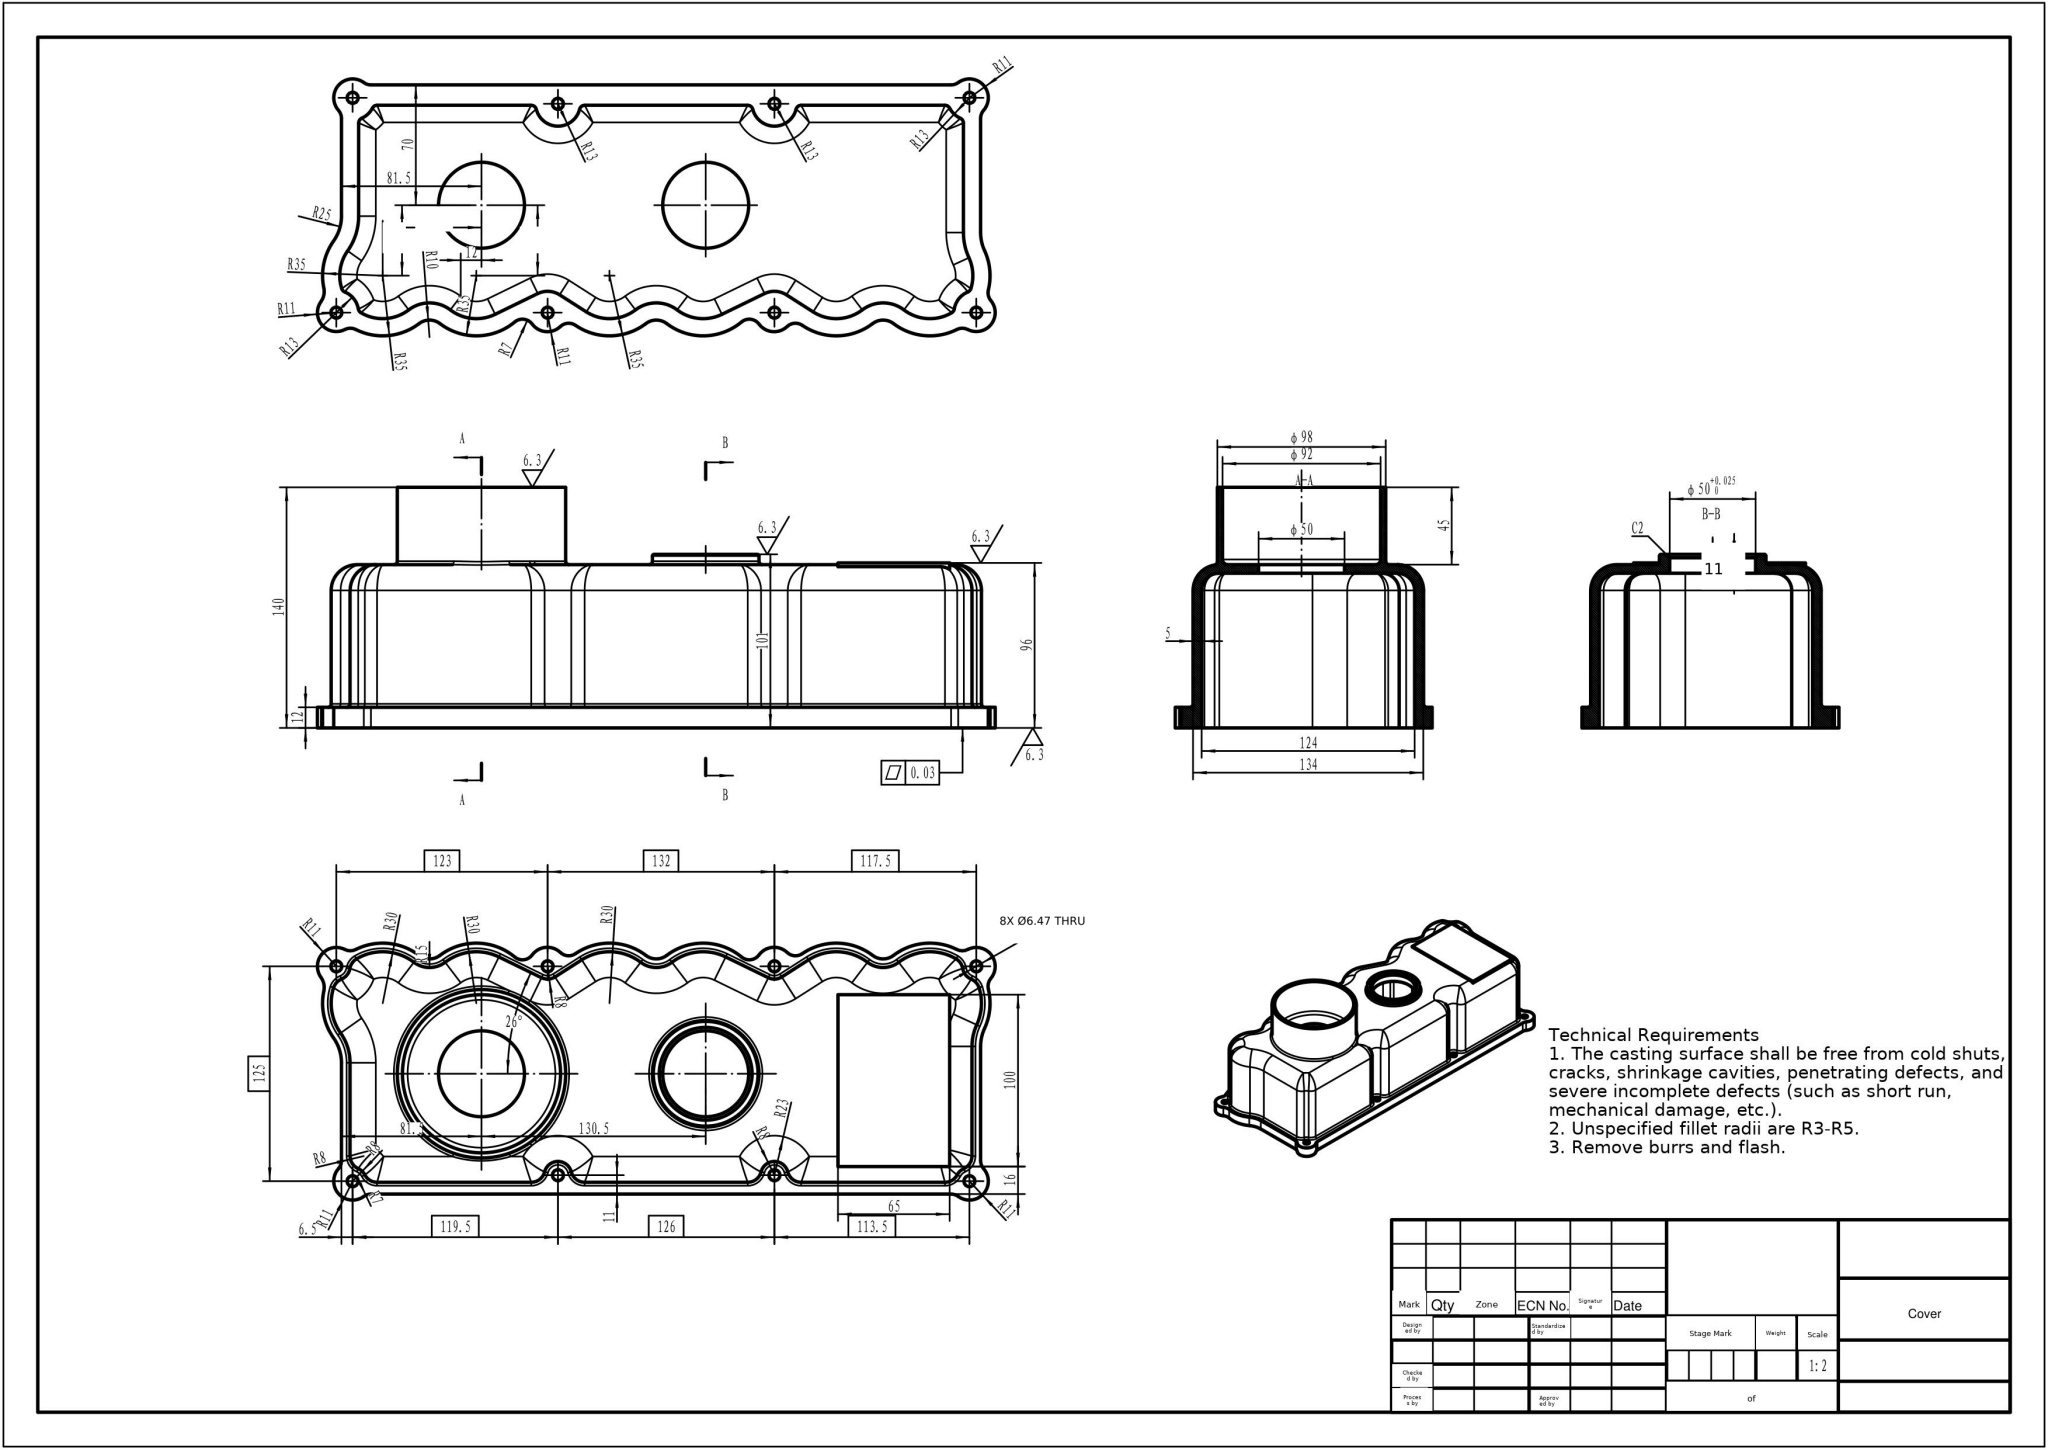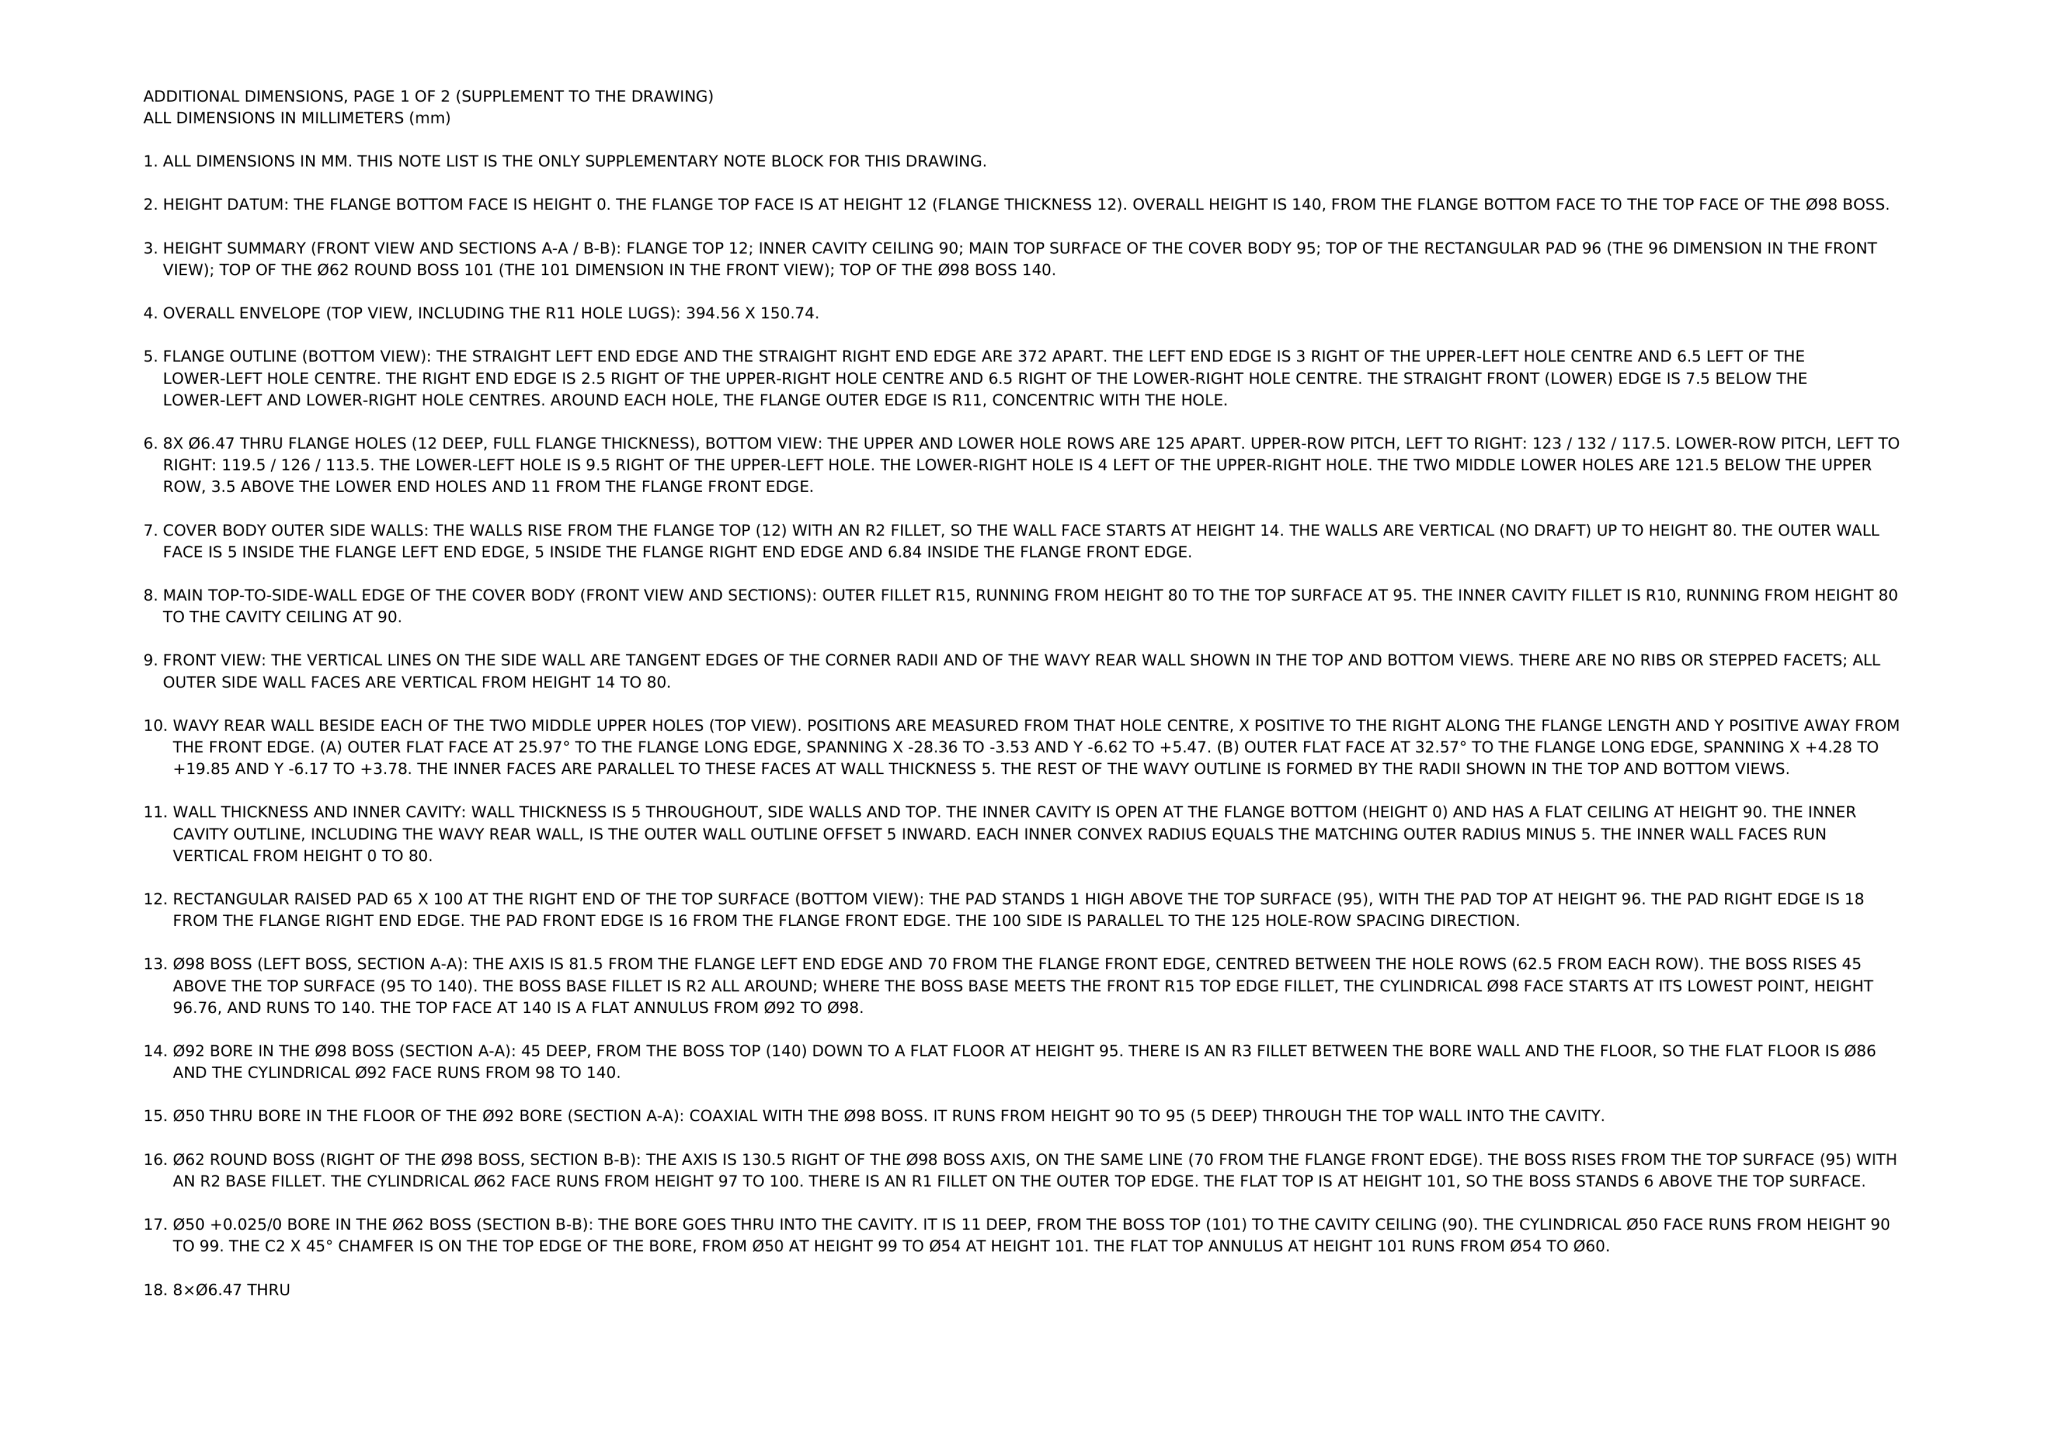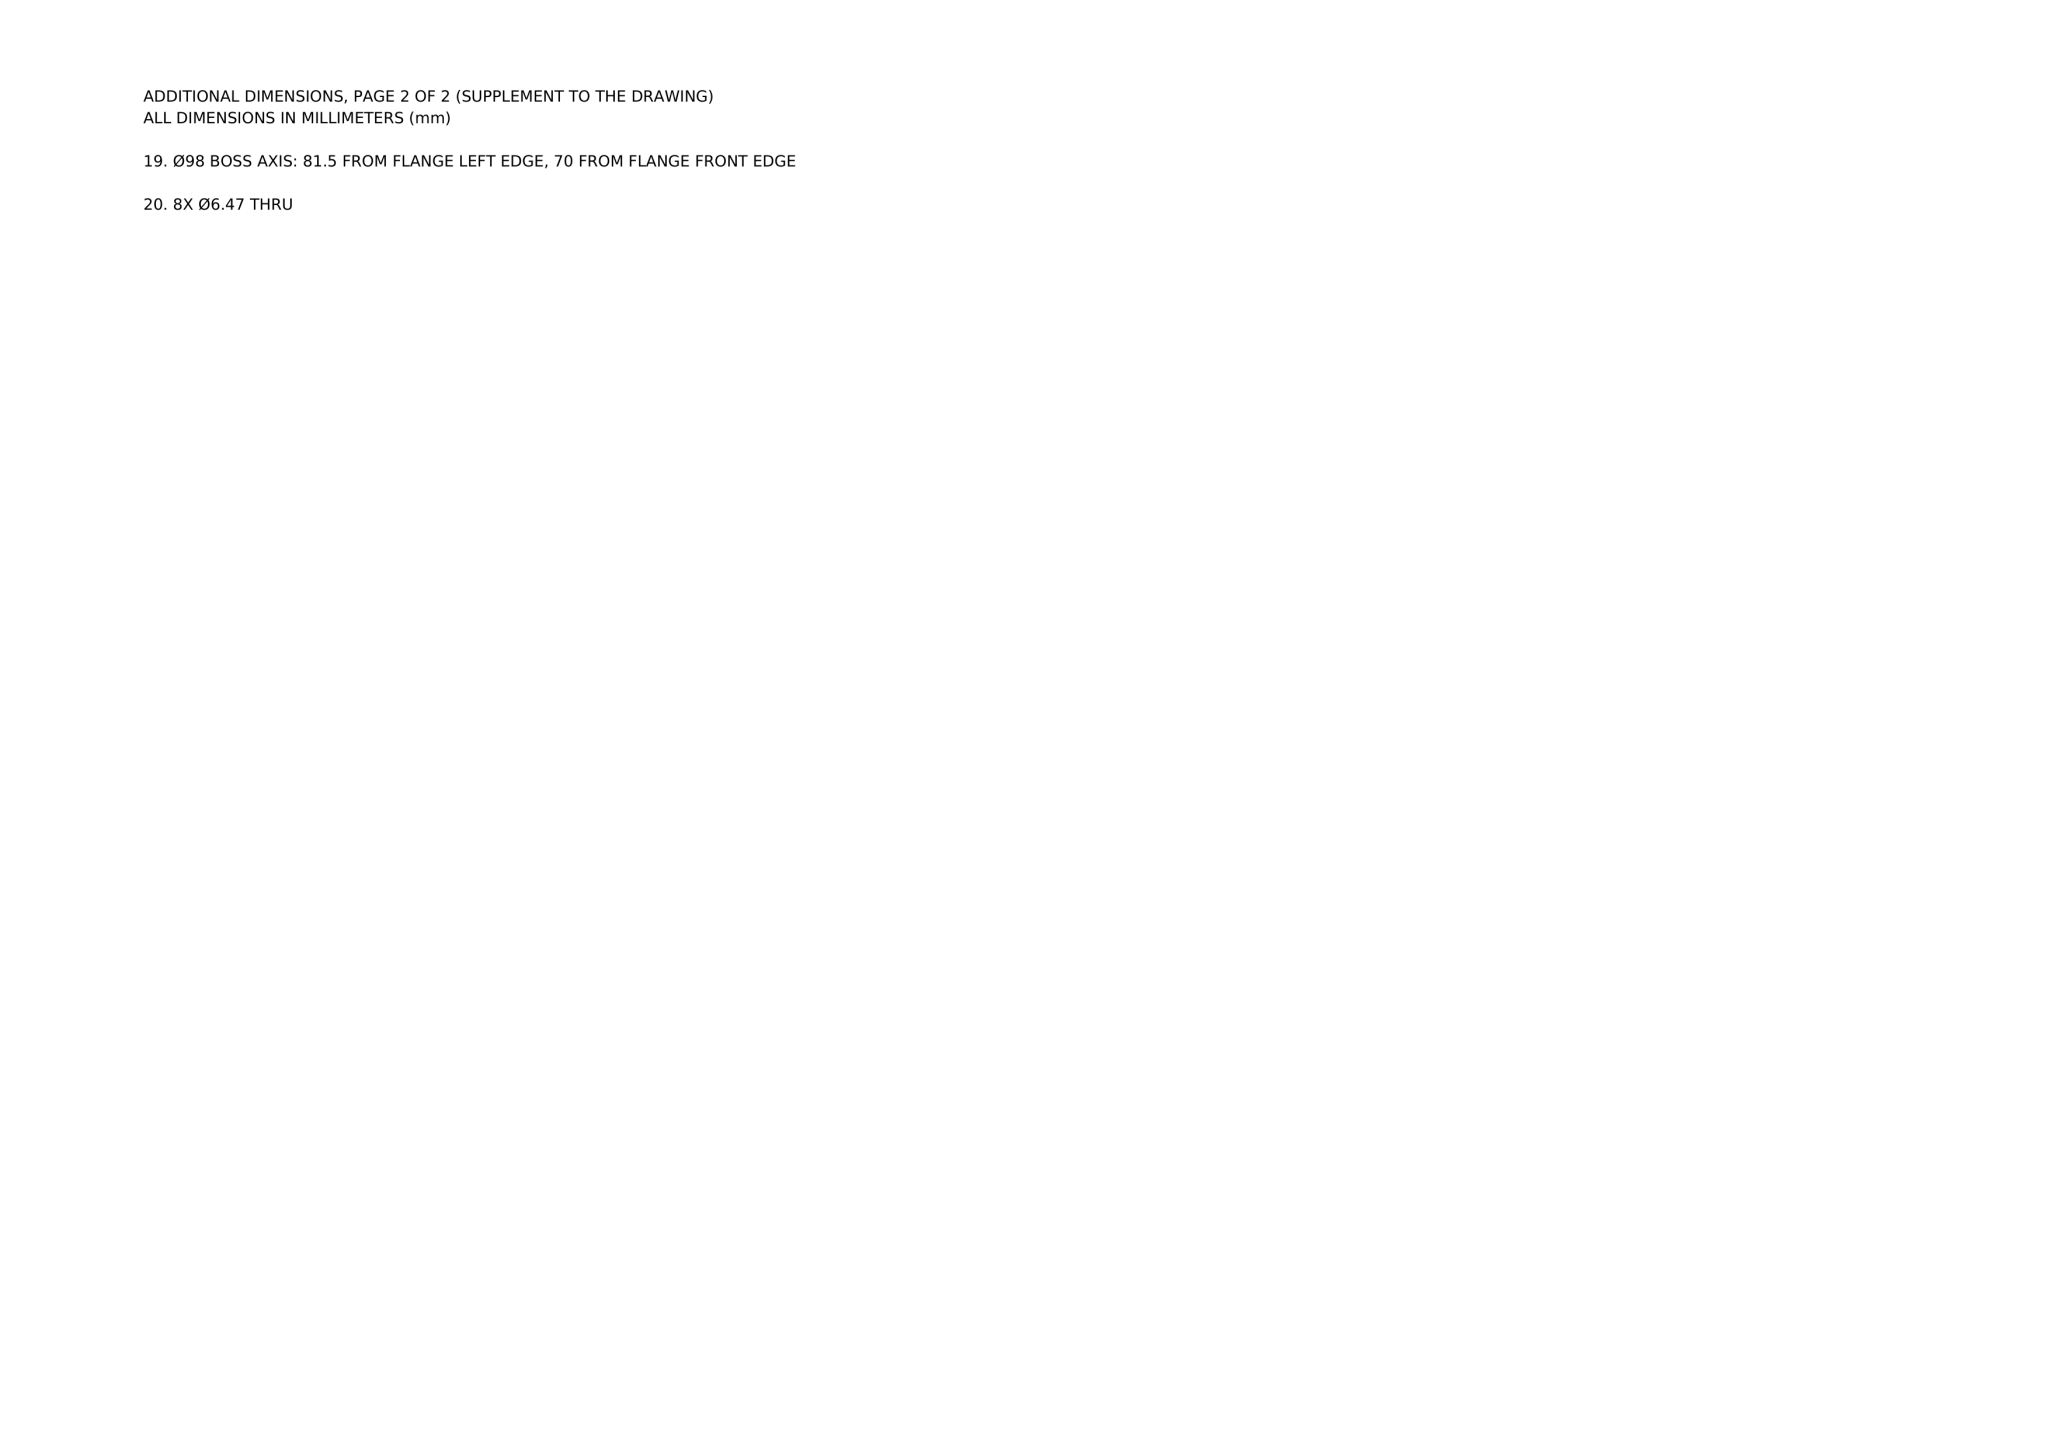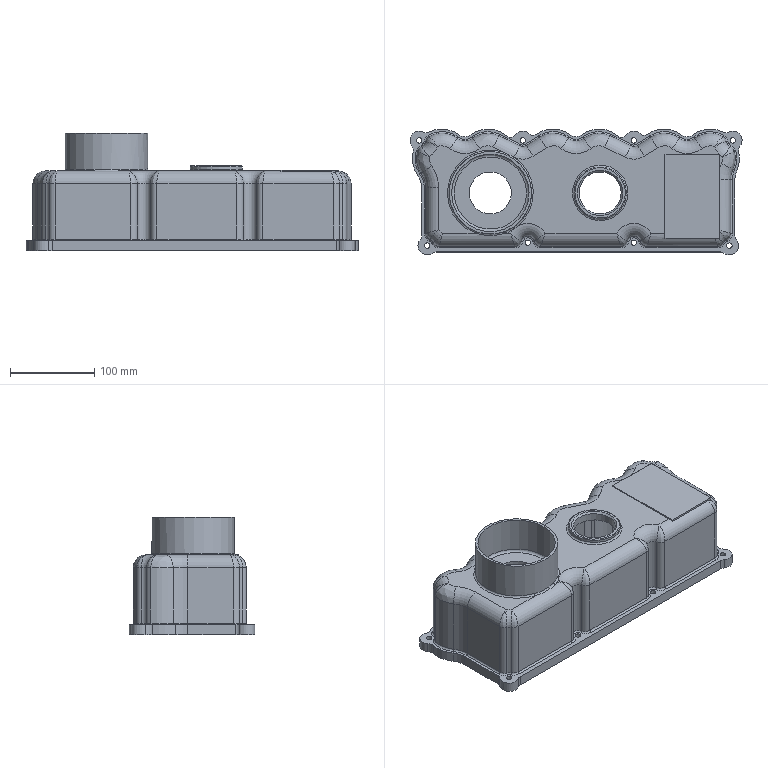Part | NX | mm | 1 solid | 282 faces | box 394.5 x 149.5 x 140 mm | volume 779138 mm3 | cylinder 137 | torus 77 | plane 36 | spline 31 | cone 1 | commonest cylinder face diameters 16 x20 20 x13 30 x12 50 x12 6 x12 14 x11 70 x10 60 x10